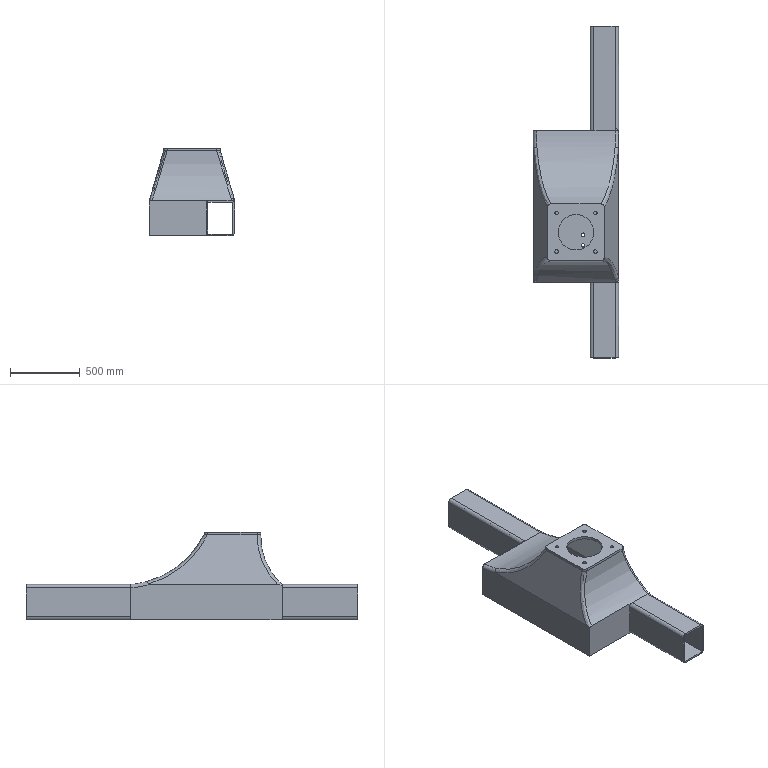Component | NX | BASE | 2 solids | 86 faces | volume 45312486 mm3 | plane 40 | cylinder 35 | spline 4 | other 4 | torus 3 | commonest cylinder face diameters 25.4 x20 50 x10 1300 x1 900 x1 1325.4 x1 925.4 x1 254 x1